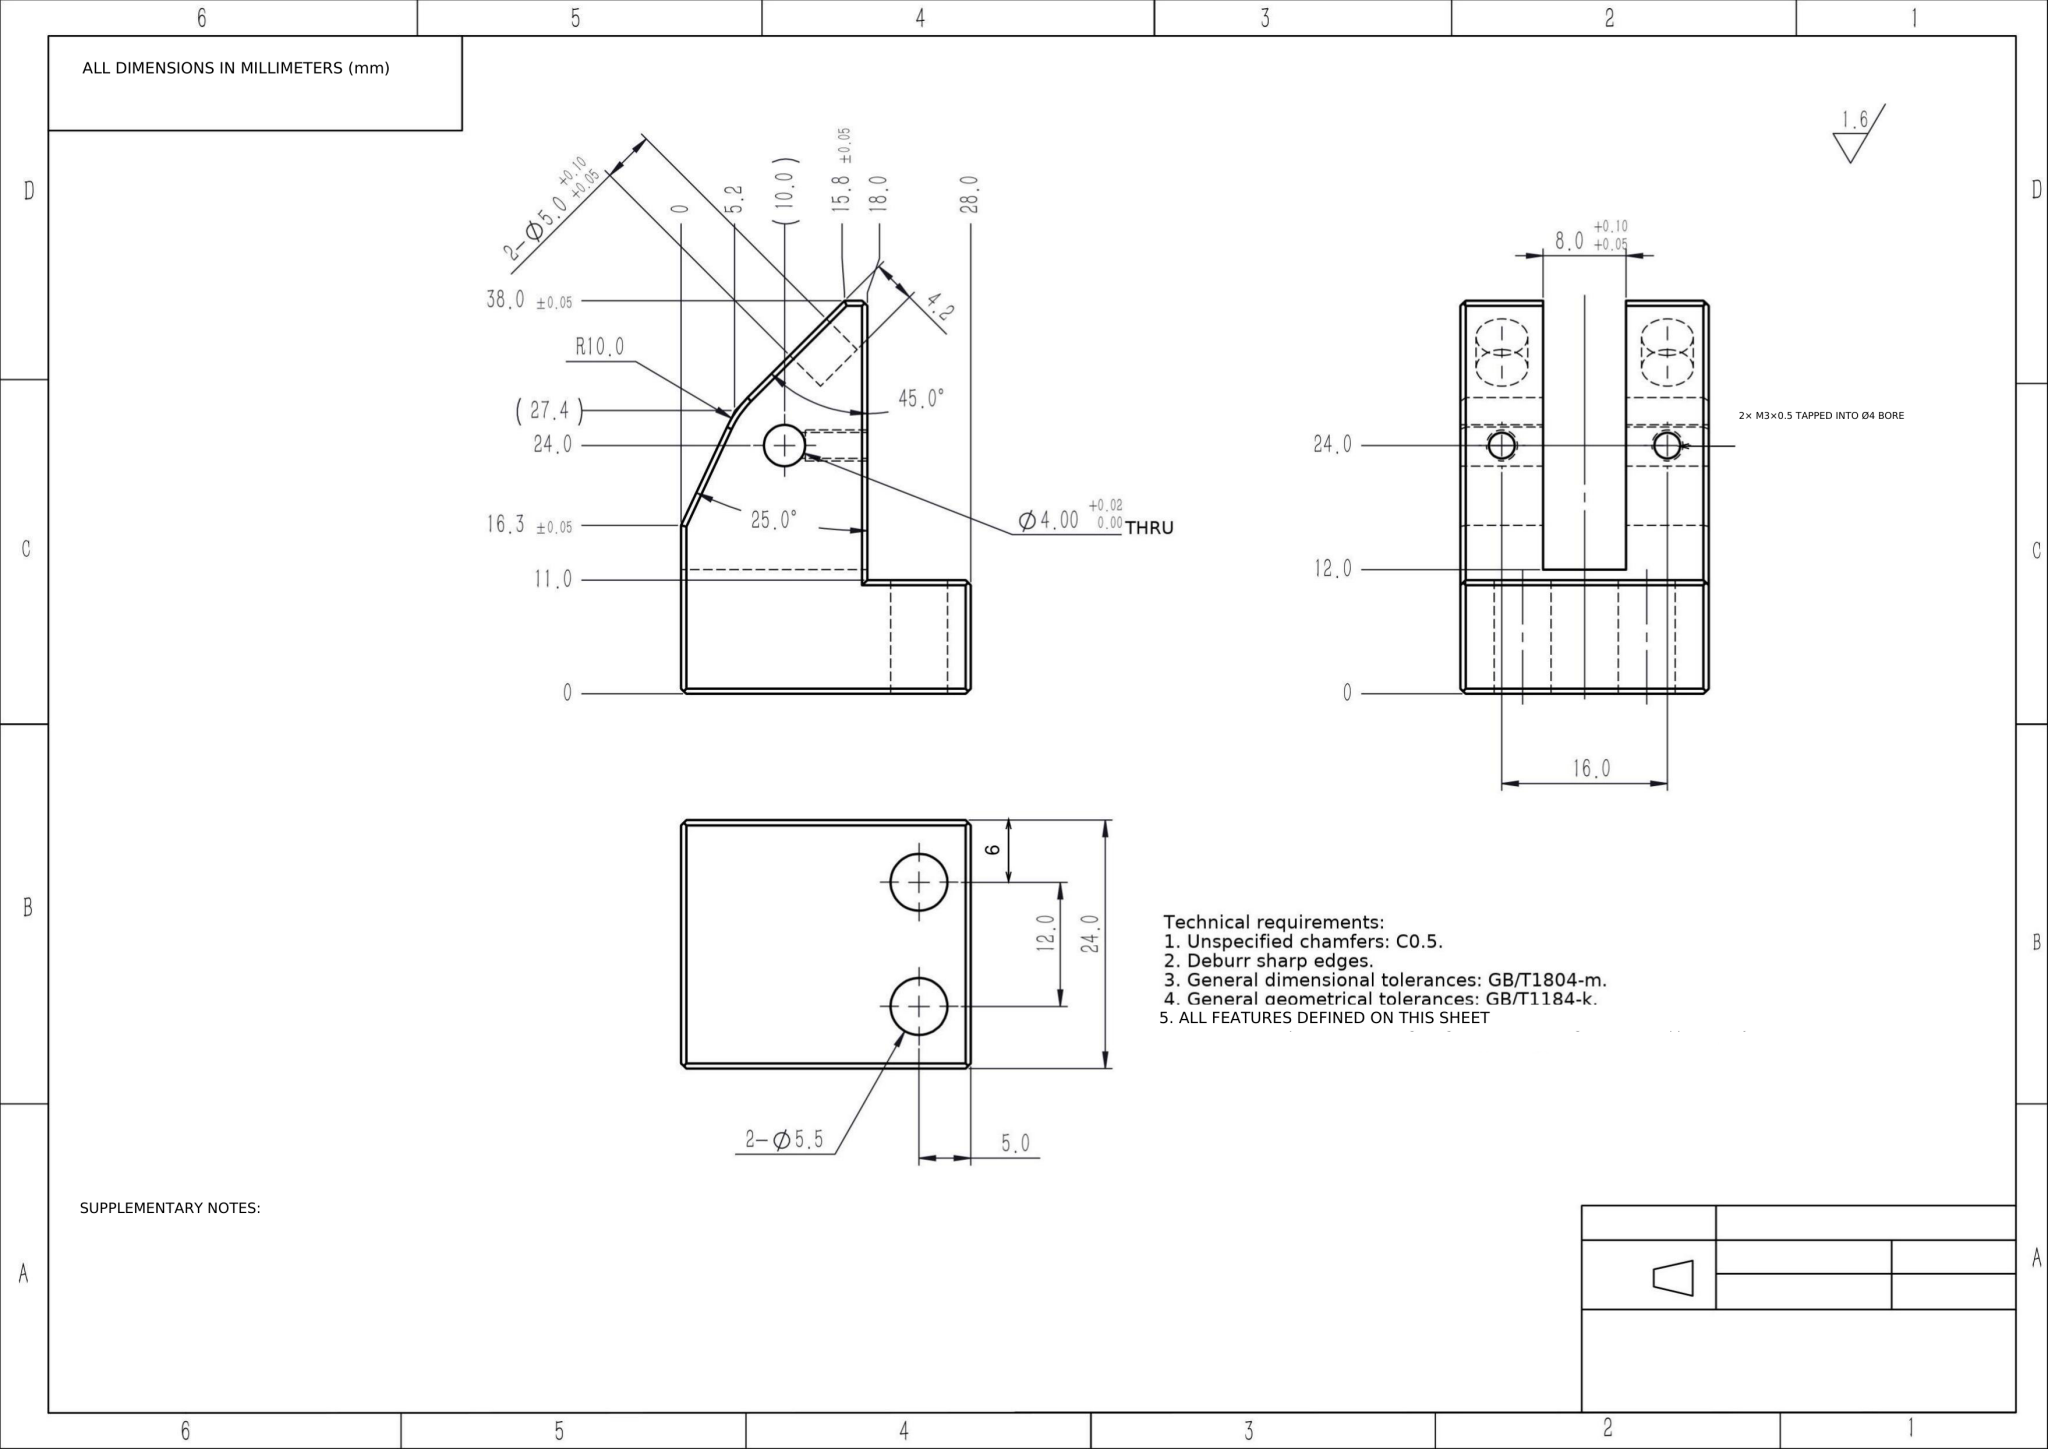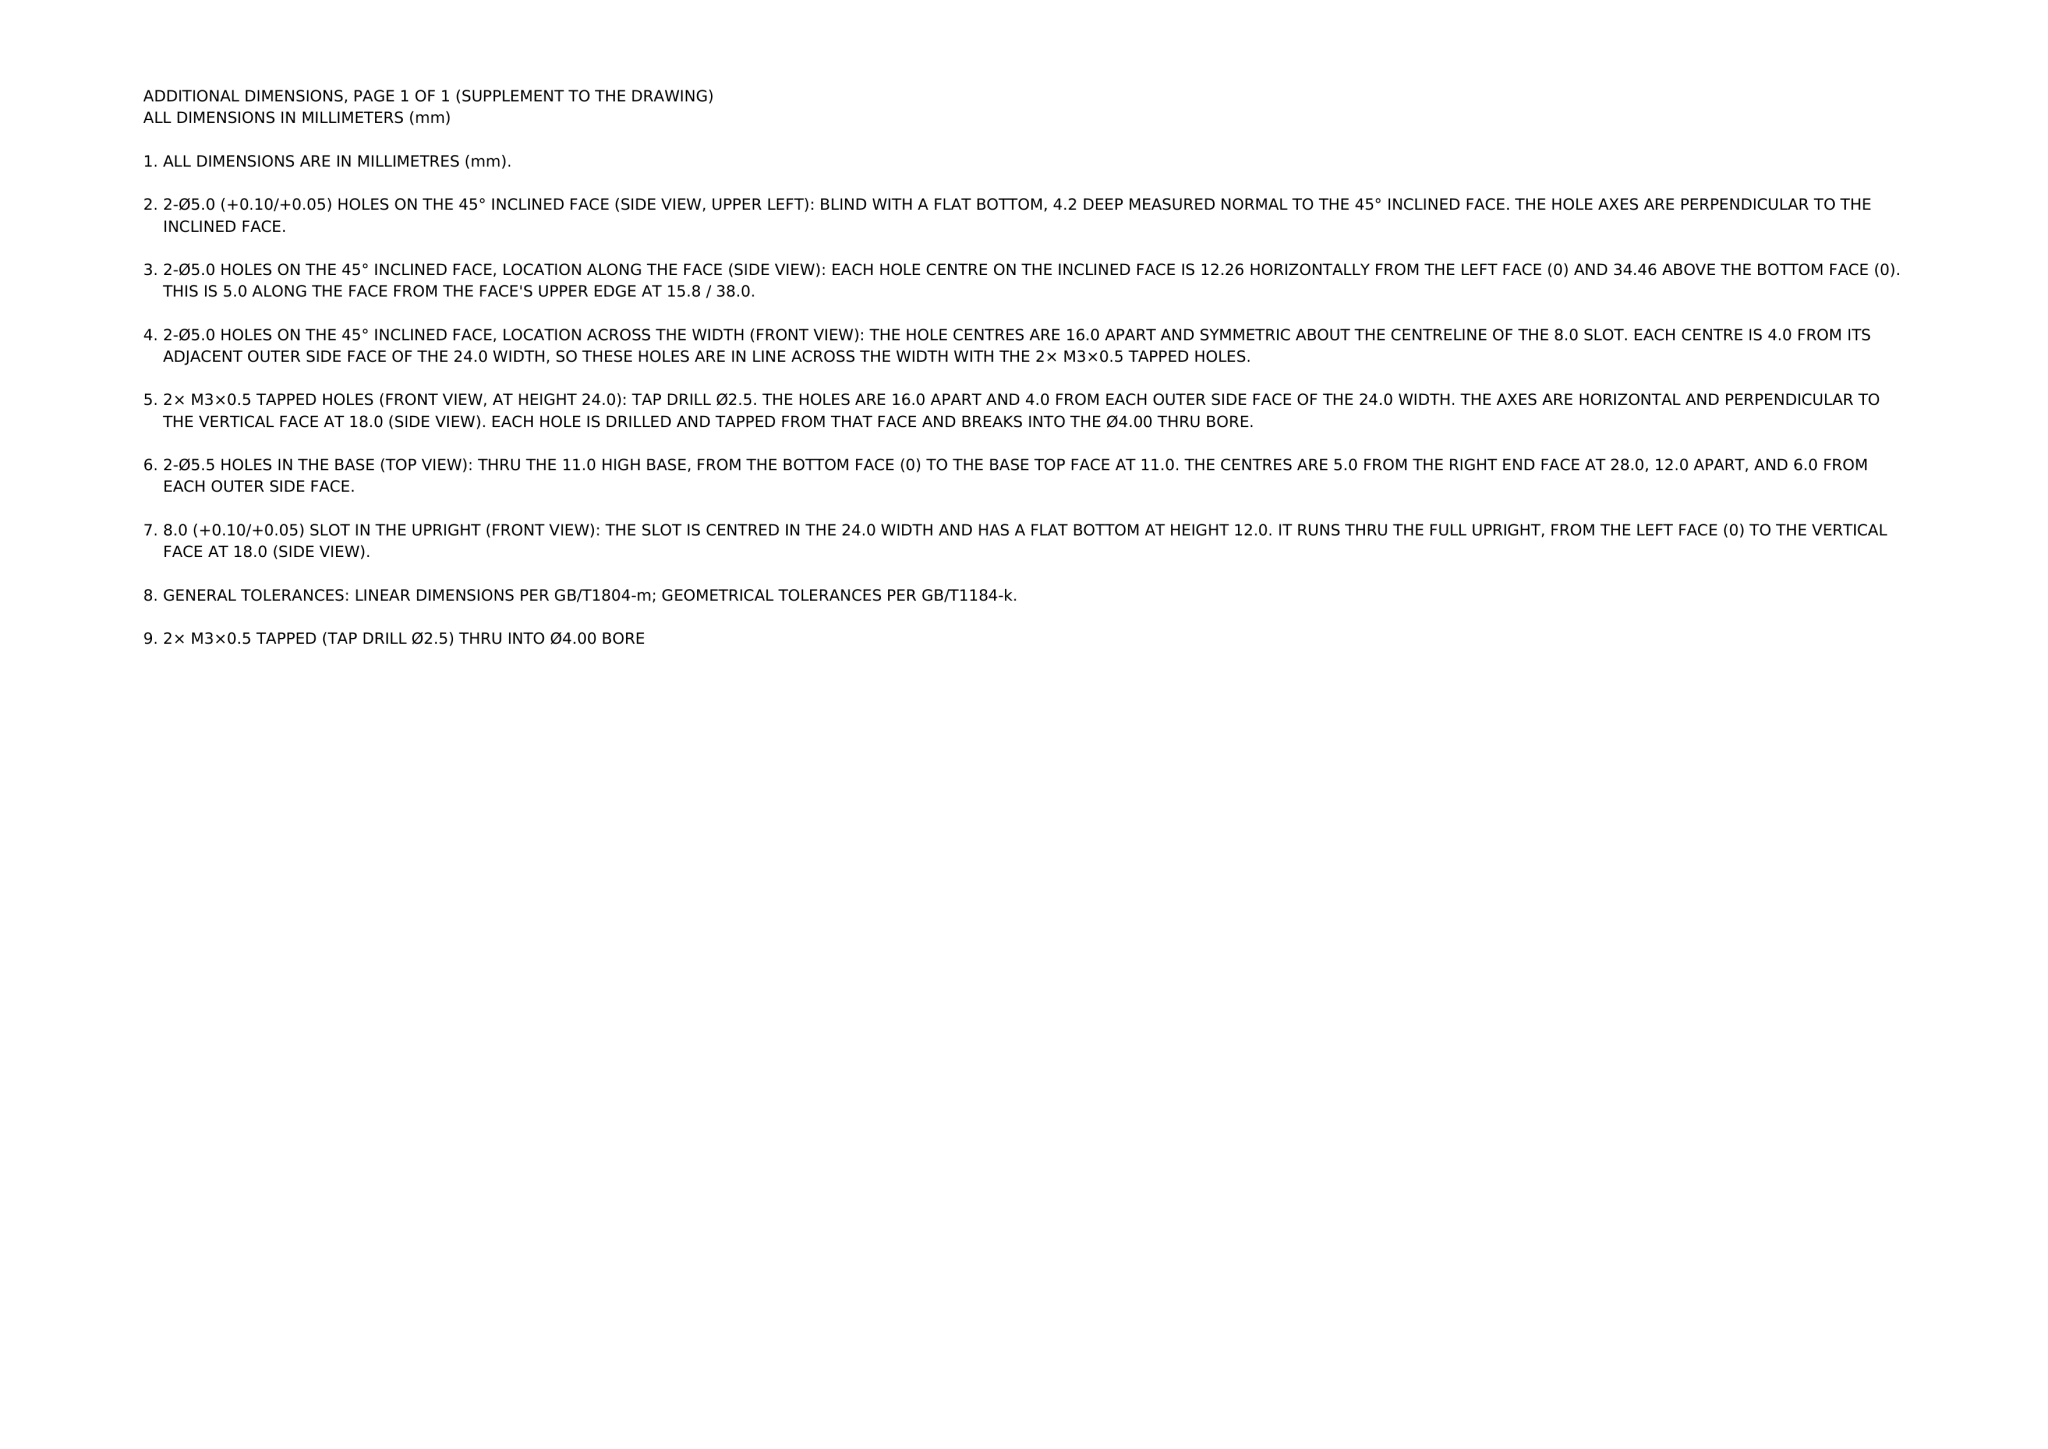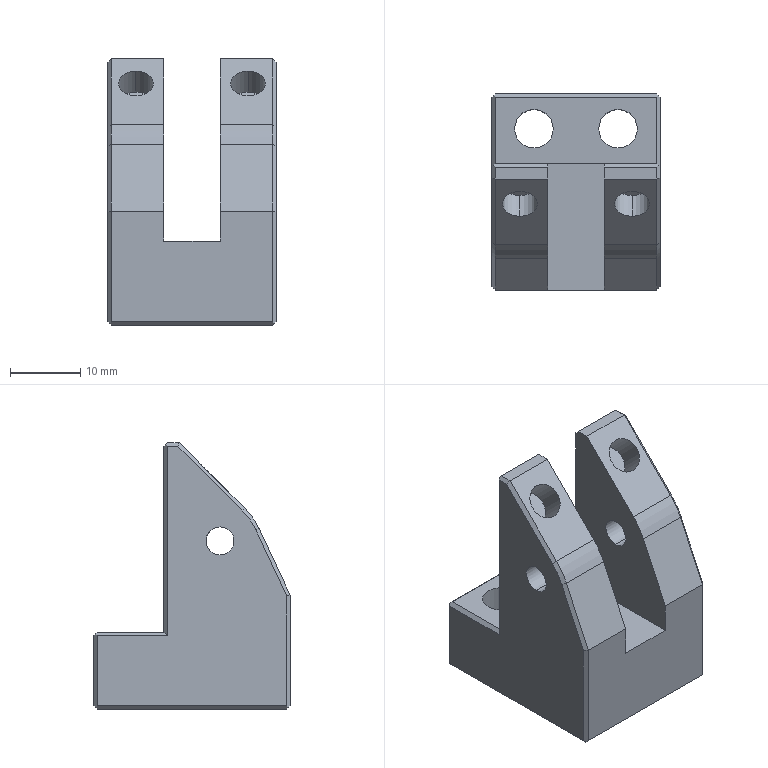Part | NX | mm | 1 solid | 59 faces | box 24 x 28 x 38 mm | volume 12078 mm3 | plane 39 | cylinder 18 | cone 2 | commonest cylinder face diameters 2.5 x4 5.5 x4 4 x4 5 x4 20 x2